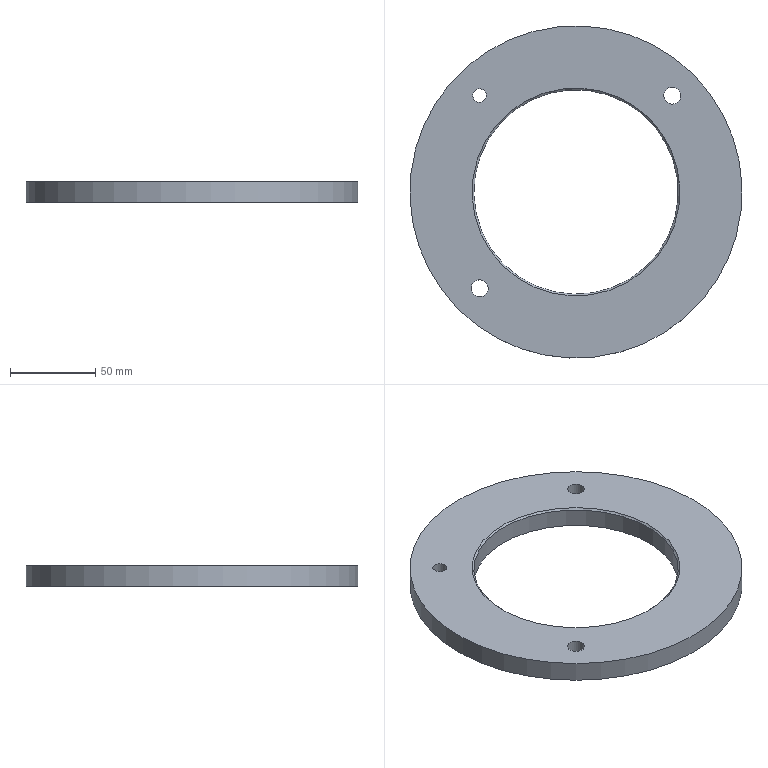Component | NX | CA6140-ZHUZHOU-YOUGAI | 1 solid | 8 faces | box 195 x 195 x 12 mm | volume 219983 mm3 | cylinder 5 | plane 2 | cone 1 | commonest cylinder face diameters 10 x2 195 x1 120 x1 8 x1
STEP:
#1=CARTESIAN_POINT('',(0.,0.,0.));
#2=DIRECTION('',(0.,0.,1.));
#3=DIRECTION('',(1.,0.,0.));
#4=AXIS2_PLACEMENT_3D('',#1,#2,#3);
#5=CARTESIAN_POINT('',(-43.134,-43.134,124.));
#6=VERTEX_POINT('',#5);
#7=CARTESIAN_POINT('',(0.,-0.,124.));
#8=DIRECTION('',(0.,0.,-1.));
#9=DIRECTION('',(-0.7071,-0.7071,0.));
#10=AXIS2_PLACEMENT_3D('',#7,#8,#9);
#11=CIRCLE('',#10,61.);
#12=CARTESIAN_POINT('',(0.,-0.,124.));
#13=DIRECTION('',(0.,0.,1.));
#14=DIRECTION('',(-0.7071,-0.7071,0.));
#15=AXIS2_PLACEMENT_3D('',#12,#13,#14);
#16=PLANE('',#15);
#17=CARTESIAN_POINT('',(61.,0.));
#18=CARTESIAN_POINT('',(61.,-105.655));
#19=CARTESIAN_POINT('',(-30.5,-52.828));
#20=CARTESIAN_POINT('',(-122.,-0.));
#21=CARTESIAN_POINT('',(-30.5,52.828));
#22=CARTESIAN_POINT('',(61.,105.655));
#23=CARTESIAN_POINT('',(61.,0.));
#24=(BOUNDED_CURVE()B_SPLINE_CURVE(2,(#17,#18,#19,#20,#21,#22,#23),.UNSPECIFIED.,.T.,.F.)B_SPLINE_CURVE_WITH_KNOTS((1,2,2,2,2,1),(-2.094,0.,2.094,4.189,6.283,8.378),.UNSPECIFIED.)CURVE()GEOMETRIC_REPRESENTATION_ITEM()RATIONAL_B_SPLINE_CURVE((1.,0.5,1.,0.5,1.,0.5,1.))REPRESENTATION_ITEM(''));
#25=(GEOMETRIC_REPRESENTATION_CONTEXT(2)PARAMETRIC_REPRESENTATION_CONTEXT()REPRESENTATION_CONTEXT('',''));
#26=DEFINITIONAL_REPRESENTATION('',(#24),#25);
#27=PCURVE('',#16,#26);
#28=CARTESIAN_POINT('',(0.,-0.,123.));
#29=DIRECTION('',(0.,0.,1.));
#30=DIRECTION('',(-0.7071,-0.7071,0.));
#31=AXIS2_PLACEMENT_3D('',#28,#29,#30);
#32=CONICAL_SURFACE('',#31,60.,0.7854);
#33=CARTESIAN_POINT('',(6.283,1.));
#34=DIRECTION('',(-1.,0.));
#35=VECTOR('',#34,1.);
#36=LINE('',#33,#35);
#37=(GEOMETRIC_REPRESENTATION_CONTEXT(2)PARAMETRIC_REPRESENTATION_CONTEXT()REPRESENTATION_CONTEXT('',''));
#38=DEFINITIONAL_REPRESENTATION('',(#36),#37);
#39=PCURVE('',#32,#38);
#40=SURFACE_CURVE('',#11,(#27,#39),.PCURVE_S1.);
#41=EDGE_CURVE('',#6,#6,#40,.T.);
#42=ORIENTED_EDGE('',*,*,#41,.T.);
#43=EDGE_LOOP('',(#42));
#44=FACE_BOUND('',#43,.T.);
#45=CARTESIAN_POINT('',(53.033,53.033,124.));
#46=VERTEX_POINT('',#45);
#47=CARTESIAN_POINT('',(56.569,56.569,124.));
#48=DIRECTION('',(0.,0.,-1.));
#49=DIRECTION('',(-0.7071,-0.7071,0.));
#50=AXIS2_PLACEMENT_3D('',#47,#48,#49);
#51=CIRCLE('',#50,5.);
#52=CARTESIAN_POINT('',(-75.,-0.));
#53=CARTESIAN_POINT('',(-75.,-8.66));
#54=CARTESIAN_POINT('',(-82.5,-4.33));
#55=CARTESIAN_POINT('',(-90.,-0.));
#56=CARTESIAN_POINT('',(-82.5,4.33));
#57=CARTESIAN_POINT('',(-75.,8.66));
#58=CARTESIAN_POINT('',(-75.,-0.));
#59=(BOUNDED_CURVE()B_SPLINE_CURVE(2,(#52,#53,#54,#55,#56,#57,#58),.UNSPECIFIED.,.T.,.F.)B_SPLINE_CURVE_WITH_KNOTS((1,2,2,2,2,1),(-2.094,0.,2.094,4.189,6.283,8.378),.UNSPECIFIED.)CURVE()GEOMETRIC_REPRESENTATION_ITEM()RATIONAL_B_SPLINE_CURVE((1.,0.5,1.,0.5,1.,0.5,1.))REPRESENTATION_ITEM(''));
#60=(GEOMETRIC_REPRESENTATION_CONTEXT(2)PARAMETRIC_REPRESENTATION_CONTEXT()REPRESENTATION_CONTEXT('',''));
#61=DEFINITIONAL_REPRESENTATION('',(#59),#60);
#62=PCURVE('',#16,#61);
#63=CARTESIAN_POINT('',(56.569,56.569,124.));
#64=DIRECTION('',(0.,0.,-1.));
#65=DIRECTION('',(0.7071,0.7071,0.));
#66=AXIS2_PLACEMENT_3D('',#63,#64,#65);
#67=CYLINDRICAL_SURFACE('',#66,5.);
#68=CARTESIAN_POINT('',(3.142,0.));
#69=DIRECTION('',(1.,0.));
#70=VECTOR('',#69,1.);
#71=LINE('',#68,#70);
#72=(GEOMETRIC_REPRESENTATION_CONTEXT(2)PARAMETRIC_REPRESENTATION_CONTEXT()REPRESENTATION_CONTEXT('',''));
#73=DEFINITIONAL_REPRESENTATION('',(#71),#72);
#74=PCURVE('',#67,#73);
#75=SURFACE_CURVE('',#51,(#62,#74),.PCURVE_S1.);
#76=EDGE_CURVE('',#46,#46,#75,.T.);
#77=ORIENTED_EDGE('',*,*,#76,.T.);
#78=EDGE_LOOP('',(#77));
#79=FACE_BOUND('',#78,.T.);
#80=CARTESIAN_POINT('',(-60.104,-60.104,124.));
#81=VERTEX_POINT('',#80);
#82=CARTESIAN_POINT('',(-56.569,-56.569,124.));
#83=DIRECTION('',(0.,0.,1.));
#84=DIRECTION('',(-0.7071,-0.7071,0.));
#85=AXIS2_PLACEMENT_3D('',#82,#83,#84);
#86=CIRCLE('',#85,5.);
#87=CARTESIAN_POINT('',(80.,-0.));
#88=DIRECTION('',(1.,0.));
#89=AXIS2_PLACEMENT_2D('',#87,#88);
#90=CIRCLE('',#89,5.);
#91=(GEOMETRIC_REPRESENTATION_CONTEXT(2)PARAMETRIC_REPRESENTATION_CONTEXT()REPRESENTATION_CONTEXT('',''));
#92=DEFINITIONAL_REPRESENTATION('',(#90),#91);
#93=PCURVE('',#16,#92);
#94=CARTESIAN_POINT('',(-56.569,-56.569,124.));
#95=DIRECTION('',(0.,0.,-1.));
#96=DIRECTION('',(0.7071,0.7071,0.));
#97=AXIS2_PLACEMENT_3D('',#94,#95,#96);
#98=CYLINDRICAL_SURFACE('',#97,5.);
#99=CARTESIAN_POINT('',(9.425,0.));
#100=DIRECTION('',(-1.,0.));
#101=VECTOR('',#100,1.);
#102=LINE('',#99,#101);
#103=(GEOMETRIC_REPRESENTATION_CONTEXT(2)PARAMETRIC_REPRESENTATION_CONTEXT()REPRESENTATION_CONTEXT('',''));
#104=DEFINITIONAL_REPRESENTATION('',(#102),#103);
#105=PCURVE('',#98,#104);
#106=SURFACE_CURVE('',#86,(#93,#105),.PCURVE_S1.);
#107=EDGE_CURVE('',#81,#81,#106,.T.);
#108=ORIENTED_EDGE('',*,*,#107,.F.);
#109=EDGE_LOOP('',(#108));
#110=FACE_BOUND('',#109,.T.);
#111=CARTESIAN_POINT('',(68.943,68.943,124.));
#112=VERTEX_POINT('',#111);
#113=CARTESIAN_POINT('',(-68.943,-68.943,124.));
#114=VERTEX_POINT('',#113);
#115=CARTESIAN_POINT('',(0.,-0.,124.));
#116=DIRECTION('',(0.,0.,-1.));
#117=DIRECTION('',(0.7071,0.7071,0.));
#118=AXIS2_PLACEMENT_3D('',#115,#116,#117);
#119=CIRCLE('',#118,97.5);
#120=CARTESIAN_POINT('',(-97.5,0.));
#121=CARTESIAN_POINT('',(-97.5,168.875));
#122=CARTESIAN_POINT('',(48.75,84.437));
#123=CARTESIAN_POINT('',(195.,0.));
#124=CARTESIAN_POINT('',(48.75,-84.437));
#125=CARTESIAN_POINT('',(-97.5,-168.875));
#126=CARTESIAN_POINT('',(-97.5,0.));
#127=(BOUNDED_CURVE()B_SPLINE_CURVE(2,(#120,#121,#122,#123,#124,#125,#126),.UNSPECIFIED.,.T.,.F.)B_SPLINE_CURVE_WITH_KNOTS((1,2,2,2,2,1),(-2.094,0.,2.094,4.189,6.283,8.378),.UNSPECIFIED.)CURVE()GEOMETRIC_REPRESENTATION_ITEM()RATIONAL_B_SPLINE_CURVE((1.,0.5,1.,0.5,1.,0.5,1.))REPRESENTATION_ITEM(''));
#128=(GEOMETRIC_REPRESENTATION_CONTEXT(2)PARAMETRIC_REPRESENTATION_CONTEXT()REPRESENTATION_CONTEXT('',''));
#129=DEFINITIONAL_REPRESENTATION('',(#127),#128);
#130=PCURVE('',#16,#129);
#131=CARTESIAN_POINT('',(0.,-0.,112.));
#132=DIRECTION('',(0.,0.,1.));
#133=DIRECTION('',(-0.7071,-0.7071,0.));
#134=AXIS2_PLACEMENT_3D('',#131,#132,#133);
#135=CYLINDRICAL_SURFACE('',#134,97.5);
#136=CARTESIAN_POINT('',(3.142,12.));
#137=DIRECTION('',(-1.,0.));
#138=VECTOR('',#137,1.);
#139=LINE('',#136,#138);
#140=(GEOMETRIC_REPRESENTATION_CONTEXT(2)PARAMETRIC_REPRESENTATION_CONTEXT()REPRESENTATION_CONTEXT('',''));
#141=DEFINITIONAL_REPRESENTATION('',(#139),#140);
#142=PCURVE('',#135,#141);
#143=SURFACE_CURVE('',#119,(#130,#142),.PCURVE_S1.);
#144=EDGE_CURVE('',#112,#114,#143,.T.);
#145=ORIENTED_EDGE('',*,*,#144,.F.);
#146=CARTESIAN_POINT('',(0.,-0.,124.));
#147=DIRECTION('',(0.,0.,-1.));
#148=DIRECTION('',(0.7071,0.7071,0.));
#149=AXIS2_PLACEMENT_3D('',#146,#147,#148);
#150=CIRCLE('',#149,97.5);
#151=CARTESIAN_POINT('',(-97.5,0.));
#152=CARTESIAN_POINT('',(-97.5,168.875));
#153=CARTESIAN_POINT('',(48.75,84.437));
#154=CARTESIAN_POINT('',(195.,0.));
#155=CARTESIAN_POINT('',(48.75,-84.437));
#156=CARTESIAN_POINT('',(-97.5,-168.875));
#157=CARTESIAN_POINT('',(-97.5,0.));
#158=(BOUNDED_CURVE()B_SPLINE_CURVE(2,(#151,#152,#153,#154,#155,#156,#157),.UNSPECIFIED.,.T.,.F.)B_SPLINE_CURVE_WITH_KNOTS((1,2,2,2,2,1),(-2.094,0.,2.094,4.189,6.283,8.378),.UNSPECIFIED.)CURVE()GEOMETRIC_REPRESENTATION_ITEM()RATIONAL_B_SPLINE_CURVE((1.,0.5,1.,0.5,1.,0.5,1.))REPRESENTATION_ITEM(''));
#159=(GEOMETRIC_REPRESENTATION_CONTEXT(2)PARAMETRIC_REPRESENTATION_CONTEXT()REPRESENTATION_CONTEXT('',''));
#160=DEFINITIONAL_REPRESENTATION('',(#158),#159);
#161=PCURVE('',#16,#160);
#162=CARTESIAN_POINT('',(9.425,12.));
#163=DIRECTION('',(-1.,0.));
#164=VECTOR('',#163,1.);
#165=LINE('',#162,#164);
#166=(GEOMETRIC_REPRESENTATION_CONTEXT(2)PARAMETRIC_REPRESENTATION_CONTEXT()REPRESENTATION_CONTEXT('',''));
#167=DEFINITIONAL_REPRESENTATION('',(#165),#166);
#168=PCURVE('',#135,#167);
#169=SURFACE_CURVE('',#150,(#161,#168),.PCURVE_S1.);
#170=EDGE_CURVE('',#114,#112,#169,.T.);
#171=ORIENTED_EDGE('',*,*,#170,.F.);
#172=EDGE_LOOP('',(#145,#171));
#173=FACE_BOUND('',#172,.T.);
#174=CARTESIAN_POINT('',(-59.397,53.74,124.));
#175=VERTEX_POINT('',#174);
#176=CARTESIAN_POINT('',(-56.569,56.569,124.));
#177=DIRECTION('',(0.,0.,-1.));
#178=DIRECTION('',(-0.7071,-0.7071,0.));
#179=AXIS2_PLACEMENT_3D('',#176,#177,#178);
#180=CIRCLE('',#179,4.);
#181=CARTESIAN_POINT('',(4.,-80.));
#182=CARTESIAN_POINT('',(4.,-86.928));
#183=CARTESIAN_POINT('',(-2.,-83.464));
#184=CARTESIAN_POINT('',(-8.,-80.));
#185=CARTESIAN_POINT('',(-2.,-76.536));
#186=CARTESIAN_POINT('',(4.,-73.072));
#187=CARTESIAN_POINT('',(4.,-80.));
#188=(BOUNDED_CURVE()B_SPLINE_CURVE(2,(#181,#182,#183,#184,#185,#186,#187),.UNSPECIFIED.,.T.,.F.)B_SPLINE_CURVE_WITH_KNOTS((1,2,2,2,2,1),(-2.094,0.,2.094,4.189,6.283,8.378),.UNSPECIFIED.)CURVE()GEOMETRIC_REPRESENTATION_ITEM()RATIONAL_B_SPLINE_CURVE((1.,0.5,1.,0.5,1.,0.5,1.))REPRESENTATION_ITEM(''));
#189=(GEOMETRIC_REPRESENTATION_CONTEXT(2)PARAMETRIC_REPRESENTATION_CONTEXT()REPRESENTATION_CONTEXT('',''));
#190=DEFINITIONAL_REPRESENTATION('',(#188),#189);
#191=PCURVE('',#16,#190);
#192=CARTESIAN_POINT('',(-56.569,56.569,124.));
#193=DIRECTION('',(0.,0.,-1.));
#194=DIRECTION('',(0.7071,0.7071,0.));
#195=AXIS2_PLACEMENT_3D('',#192,#193,#194);
#196=CYLINDRICAL_SURFACE('',#195,4.);
#197=CARTESIAN_POINT('',(3.142,0.));
#198=DIRECTION('',(1.,0.));
#199=VECTOR('',#198,1.);
#200=LINE('',#197,#199);
#201=(GEOMETRIC_REPRESENTATION_CONTEXT(2)PARAMETRIC_REPRESENTATION_CONTEXT()REPRESENTATION_CONTEXT('',''));
#202=DEFINITIONAL_REPRESENTATION('',(#200),#201);
#203=PCURVE('',#196,#202);
#204=SURFACE_CURVE('',#180,(#191,#203),.PCURVE_S1.);
#205=EDGE_CURVE('',#175,#175,#204,.T.);
#206=ORIENTED_EDGE('',*,*,#205,.T.);
#207=EDGE_LOOP('',(#206));
#208=FACE_BOUND('',#207,.T.);
#209=ADVANCED_FACE('',(#44,#79,#110,#173,#208),#16,.T.);
#210=CARTESIAN_POINT('',(-59.397,53.74,112.));
#211=VERTEX_POINT('',#210);
#212=CARTESIAN_POINT('',(-56.569,56.569,112.));
#213=DIRECTION('',(0.,0.,-1.));
#214=DIRECTION('',(-0.7071,-0.7071,0.));
#215=AXIS2_PLACEMENT_3D('',#212,#213,#214);
#216=CIRCLE('',#215,4.);
#217=CARTESIAN_POINT('',(0.,-0.,112.));
#218=DIRECTION('',(0.,0.,-1.));
#219=DIRECTION('',(0.7071,0.7071,0.));
#220=AXIS2_PLACEMENT_3D('',#217,#218,#219);
#221=PLANE('',#220);
#222=CARTESIAN_POINT('',(0.,-80.));
#223=DIRECTION('',(-1.,0.));
#224=AXIS2_PLACEMENT_2D('',#222,#223);
#225=CIRCLE('',#224,4.);
#226=(GEOMETRIC_REPRESENTATION_CONTEXT(2)PARAMETRIC_REPRESENTATION_CONTEXT()REPRESENTATION_CONTEXT('',''));
#227=DEFINITIONAL_REPRESENTATION('',(#225),#226);
#228=PCURVE('',#221,#227);
#229=CARTESIAN_POINT('',(3.142,12.));
#230=DIRECTION('',(1.,0.));
#231=VECTOR('',#230,1.);
#232=LINE('',#229,#231);
#233=(GEOMETRIC_REPRESENTATION_CONTEXT(2)PARAMETRIC_REPRESENTATION_CONTEXT()REPRESENTATION_CONTEXT('',''));
#234=DEFINITIONAL_REPRESENTATION('',(#232),#233);
#235=PCURVE('',#196,#234);
#236=SURFACE_CURVE('',#216,(#228,#235),.PCURVE_S1.);
#237=EDGE_CURVE('',#211,#211,#236,.T.);
#238=ORIENTED_EDGE('',*,*,#237,.F.);
#239=EDGE_LOOP('',(#238));
#240=FACE_BOUND('',#239,.T.);
#241=CARTESIAN_POINT('',(53.033,53.033,112.));
#242=VERTEX_POINT('',#241);
#243=CARTESIAN_POINT('',(56.569,56.569,112.));
#244=DIRECTION('',(0.,0.,-1.));
#245=DIRECTION('',(-0.7071,-0.7071,0.));
#246=AXIS2_PLACEMENT_3D('',#243,#244,#245);
#247=CIRCLE('',#246,5.);
#248=CARTESIAN_POINT('',(80.,-0.));
#249=DIRECTION('',(-1.,0.));
#250=AXIS2_PLACEMENT_2D('',#248,#249);
#251=CIRCLE('',#250,5.);
#252=(GEOMETRIC_REPRESENTATION_CONTEXT(2)PARAMETRIC_REPRESENTATION_CONTEXT()REPRESENTATION_CONTEXT('',''));
#253=DEFINITIONAL_REPRESENTATION('',(#251),#252);
#254=PCURVE('',#221,#253);
#255=CARTESIAN_POINT('',(3.142,12.));
#256=DIRECTION('',(1.,0.));
#257=VECTOR('',#256,1.);
#258=LINE('',#255,#257);
#259=(GEOMETRIC_REPRESENTATION_CONTEXT(2)PARAMETRIC_REPRESENTATION_CONTEXT()REPRESENTATION_CONTEXT('',''));
#260=DEFINITIONAL_REPRESENTATION('',(#258),#259);
#261=PCURVE('',#67,#260);
#262=SURFACE_CURVE('',#247,(#254,#261),.PCURVE_S1.);
#263=EDGE_CURVE('',#242,#242,#262,.T.);
#264=ORIENTED_EDGE('',*,*,#263,.F.);
#265=EDGE_LOOP('',(#264));
#266=FACE_BOUND('',#265,.T.);
#267=CARTESIAN_POINT('',(-68.943,-68.943,112.));
#268=VERTEX_POINT('',#267);
#269=CARTESIAN_POINT('',(0.,-0.,112.));
#270=DIRECTION('',(0.,0.,1.));
#271=DIRECTION('',(-0.7071,-0.7071,0.));
#272=AXIS2_PLACEMENT_3D('',#269,#270,#271);
#273=CIRCLE('',#272,97.5);
#274=CARTESIAN_POINT('',(-97.5,0.));
#275=CARTESIAN_POINT('',(-97.5,168.875));
#276=CARTESIAN_POINT('',(48.75,84.437));
#277=CARTESIAN_POINT('',(195.,0.));
#278=CARTESIAN_POINT('',(48.75,-84.437));
#279=CARTESIAN_POINT('',(-97.5,-168.875));
#280=CARTESIAN_POINT('',(-97.5,0.));
#281=(BOUNDED_CURVE()B_SPLINE_CURVE(2,(#274,#275,#276,#277,#278,#279,#280),.UNSPECIFIED.,.T.,.F.)B_SPLINE_CURVE_WITH_KNOTS((1,2,2,2,2,1),(-2.094,0.,2.094,4.189,6.283,8.378),.UNSPECIFIED.)CURVE()GEOMETRIC_REPRESENTATION_ITEM()RATIONAL_B_SPLINE_CURVE((1.,0.5,1.,0.5,1.,0.5,1.))REPRESENTATION_ITEM(''));
#282=(GEOMETRIC_REPRESENTATION_CONTEXT(2)PARAMETRIC_REPRESENTATION_CONTEXT()REPRESENTATION_CONTEXT('',''));
#283=DEFINITIONAL_REPRESENTATION('',(#281),#282);
#284=PCURVE('',#221,#283);
#285=CARTESIAN_POINT('',(0.,0.));
#286=DIRECTION('',(1.,0.));
#287=VECTOR('',#286,1.);
#288=LINE('',#285,#287);
#289=(GEOMETRIC_REPRESENTATION_CONTEXT(2)PARAMETRIC_REPRESENTATION_CONTEXT()REPRESENTATION_CONTEXT('',''));
#290=DEFINITIONAL_REPRESENTATION('',(#288),#289);
#291=PCURVE('',#135,#290);
#292=SURFACE_CURVE('',#273,(#284,#291),.PCURVE_S1.);
#293=EDGE_CURVE('',#268,#268,#292,.T.);
#294=ORIENTED_EDGE('',*,*,#293,.F.);
#295=EDGE_LOOP('',(#294));
#296=FACE_BOUND('',#295,.T.);
#297=CARTESIAN_POINT('',(-42.426,-42.426,112.));
#298=VERTEX_POINT('',#297);
#299=CARTESIAN_POINT('',(0.,-0.,112.));
#300=DIRECTION('',(0.,0.,1.));
#301=DIRECTION('',(-0.7071,-0.7071,0.));
#302=AXIS2_PLACEMENT_3D('',#299,#300,#301);
#303=CIRCLE('',#302,60.);
#304=CARTESIAN_POINT('',(-60.,0.));
#305=CARTESIAN_POINT('',(-60.,103.923));
#306=CARTESIAN_POINT('',(30.,51.962));
#307=CARTESIAN_POINT('',(120.,0.));
#308=CARTESIAN_POINT('',(30.,-51.962));
#309=CARTESIAN_POINT('',(-60.,-103.923));
#310=CARTESIAN_POINT('',(-60.,0.));
#311=(BOUNDED_CURVE()B_SPLINE_CURVE(2,(#304,#305,#306,#307,#308,#309,#310),.UNSPECIFIED.,.T.,.F.)B_SPLINE_CURVE_WITH_KNOTS((1,2,2,2,2,1),(-2.094,0.,2.094,4.189,6.283,8.378),.UNSPECIFIED.)CURVE()GEOMETRIC_REPRESENTATION_ITEM()RATIONAL_B_SPLINE_CURVE((1.,0.5,1.,0.5,1.,0.5,1.))REPRESENTATION_ITEM(''));
#312=(GEOMETRIC_REPRESENTATION_CONTEXT(2)PARAMETRIC_REPRESENTATION_CONTEXT()REPRESENTATION_CONTEXT('',''));
#313=DEFINITIONAL_REPRESENTATION('',(#311),#312);
#314=PCURVE('',#221,#313);
#315=CARTESIAN_POINT('',(0.,-0.,112.));
#316=DIRECTION('',(0.,0.,1.));
#317=DIRECTION('',(-0.7071,-0.7071,0.));
#318=AXIS2_PLACEMENT_3D('',#315,#316,#317);
#319=CYLINDRICAL_SURFACE('',#318,60.);
#320=CARTESIAN_POINT('',(0.,0.));
#321=DIRECTION('',(1.,0.));
#322=VECTOR('',#321,1.);
#323=LINE('',#320,#322);
#324=(GEOMETRIC_REPRESENTATION_CONTEXT(2)PARAMETRIC_REPRESENTATION_CONTEXT()REPRESENTATION_CONTEXT('',''));
#325=DEFINITIONAL_REPRESENTATION('',(#323),#324);
#326=PCURVE('',#319,#325);
#327=SURFACE_CURVE('',#303,(#314,#326),.PCURVE_S1.);
#328=EDGE_CURVE('',#298,#298,#327,.T.);
#329=ORIENTED_EDGE('',*,*,#328,.T.);
#330=EDGE_LOOP('',(#329));
#331=FACE_BOUND('',#330,.T.);
#332=CARTESIAN_POINT('',(-60.104,-60.104,112.));
#333=VERTEX_POINT('',#332);
#334=CARTESIAN_POINT('',(-56.569,-56.569,112.));
#335=DIRECTION('',(0.,0.,1.));
#336=DIRECTION('',(-0.7071,-0.7071,0.));
#337=AXIS2_PLACEMENT_3D('',#334,#335,#336);
#338=CIRCLE('',#337,5.);
#339=CARTESIAN_POINT('',(-85.,-0.));
#340=CARTESIAN_POINT('',(-85.,8.66));
#341=CARTESIAN_POINT('',(-77.5,4.33));
#342=CARTESIAN_POINT('',(-70.,-0.));
#343=CARTESIAN_POINT('',(-77.5,-4.33));
#344=CARTESIAN_POINT('',(-85.,-8.66));
#345=CARTESIAN_POINT('',(-85.,-0.));
#346=(BOUNDED_CURVE()B_SPLINE_CURVE(2,(#339,#340,#341,#342,#343,#344,#345),.UNSPECIFIED.,.T.,.F.)B_SPLINE_CURVE_WITH_KNOTS((1,2,2,2,2,1),(-2.094,0.,2.094,4.189,6.283,8.378),.UNSPECIFIED.)CURVE()GEOMETRIC_REPRESENTATION_ITEM()RATIONAL_B_SPLINE_CURVE((1.,0.5,1.,0.5,1.,0.5,1.))REPRESENTATION_ITEM(''));
#347=(GEOMETRIC_REPRESENTATION_CONTEXT(2)PARAMETRIC_REPRESENTATION_CONTEXT()REPRESENTATION_CONTEXT('',''));
#348=DEFINITIONAL_REPRESENTATION('',(#346),#347);
#349=PCURVE('',#221,#348);
#350=CARTESIAN_POINT('',(9.425,12.));
#351=DIRECTION('',(-1.,0.));
#352=VECTOR('',#351,1.);
#353=LINE('',#350,#352);
#354=(GEOMETRIC_REPRESENTATION_CONTEXT(2)PARAMETRIC_REPRESENTATION_CONTEXT()REPRESENTATION_CONTEXT('',''));
#355=DEFINITIONAL_REPRESENTATION('',(#353),#354);
#356=PCURVE('',#98,#355);
#357=SURFACE_CURVE('',#338,(#349,#356),.PCURVE_S1.);
#358=EDGE_CURVE('',#333,#333,#357,.T.);
#359=ORIENTED_EDGE('',*,*,#358,.T.);
#360=EDGE_LOOP('',(#359));
#361=FACE_BOUND('',#360,.T.);
#362=ADVANCED_FACE('',(#240,#266,#296,#331,#361),#221,.T.);
#363=ORIENTED_EDGE('',*,*,#144,.T.);
#364=CARTESIAN_POINT('',(-68.943,-68.943,112.));
#365=CARTESIAN_POINT('',(-68.943,-68.943,124.));
#366=B_SPLINE_CURVE_WITH_KNOTS('',1,(#364,#365),.UNSPECIFIED.,.F.,.F.,(2,2),(0.,12.),.PIECEWISE_BEZIER_KNOTS.);
#367=CARTESIAN_POINT('',(0.,0.));
#368=DIRECTION('',(0.,1.));
#369=VECTOR('',#368,1.);
#370=LINE('',#367,#369);
#371=(GEOMETRIC_REPRESENTATION_CONTEXT(2)PARAMETRIC_REPRESENTATION_CONTEXT()REPRESENTATION_CONTEXT('',''));
#372=DEFINITIONAL_REPRESENTATION('',(#370),#371);
#373=PCURVE('',#135,#372);
#374=CARTESIAN_POINT('',(6.283,0.));
#375=DIRECTION('',(0.,1.));
#376=VECTOR('',#375,1.);
#377=LINE('',#374,#376);
#378=(GEOMETRIC_REPRESENTATION_CONTEXT(2)PARAMETRIC_REPRESENTATION_CONTEXT()REPRESENTATION_CONTEXT('',''));
#379=DEFINITIONAL_REPRESENTATION('',(#377),#378);
#380=PCURVE('',#135,#379);
#381=SEAM_CURVE('',#366,(#373,#380),.PCURVE_S1.);
#382=EDGE_CURVE('',#268,#114,#381,.T.);
#383=ORIENTED_EDGE('',*,*,#382,.F.);
#384=ORIENTED_EDGE('',*,*,#293,.T.);
#385=ORIENTED_EDGE('',*,*,#382,.T.);
#386=ORIENTED_EDGE('',*,*,#170,.T.);
#387=EDGE_LOOP('',(#363,#383,#384,#385,#386));
#388=FACE_BOUND('',#387,.T.);
#389=ADVANCED_FACE('',(#388),#135,.T.);
#390=CARTESIAN_POINT('',(-42.426,-42.426,123.));
#391=VERTEX_POINT('',#390);
#392=CARTESIAN_POINT('',(0.,-0.,123.));
#393=DIRECTION('',(0.,0.,1.));
#394=DIRECTION('',(-0.7071,-0.7071,0.));
#395=AXIS2_PLACEMENT_3D('',#392,#393,#394);
#396=CIRCLE('',#395,60.);
#397=CARTESIAN_POINT('',(0.,11.));
#398=DIRECTION('',(1.,0.));
#399=VECTOR('',#398,1.);
#400=LINE('',#397,#399);
#401=(GEOMETRIC_REPRESENTATION_CONTEXT(2)PARAMETRIC_REPRESENTATION_CONTEXT()REPRESENTATION_CONTEXT('',''));
#402=DEFINITIONAL_REPRESENTATION('',(#400),#401);
#403=PCURVE('',#319,#402);
#404=CARTESIAN_POINT('',(0.,0.));
#405=DIRECTION('',(1.,0.));
#406=VECTOR('',#405,1.);
#407=LINE('',#404,#406);
#408=(GEOMETRIC_REPRESENTATION_CONTEXT(2)PARAMETRIC_REPRESENTATION_CONTEXT()REPRESENTATION_CONTEXT('',''));
#409=DEFINITIONAL_REPRESENTATION('',(#407),#408);
#410=PCURVE('',#32,#409);
#411=SURFACE_CURVE('',#396,(#403,#410),.PCURVE_S1.);
#412=EDGE_CURVE('',#391,#391,#411,.T.);
#413=ORIENTED_EDGE('',*,*,#412,.F.);
#414=CARTESIAN_POINT('',(-42.426,-42.426,112.));
#415=CARTESIAN_POINT('',(-42.426,-42.426,123.));
#416=B_SPLINE_CURVE_WITH_KNOTS('',1,(#414,#415),.UNSPECIFIED.,.F.,.F.,(2,2),(0.,11.),.PIECEWISE_BEZIER_KNOTS.);
#417=CARTESIAN_POINT('',(0.,0.));
#418=DIRECTION('',(0.,1.));
#419=VECTOR('',#418,1.);
#420=LINE('',#417,#419);
#421=(GEOMETRIC_REPRESENTATION_CONTEXT(2)PARAMETRIC_REPRESENTATION_CONTEXT()REPRESENTATION_CONTEXT('',''));
#422=DEFINITIONAL_REPRESENTATION('',(#420),#421);
#423=PCURVE('',#319,#422);
#424=CARTESIAN_POINT('',(6.283,0.));
#425=DIRECTION('',(0.,1.));
#426=VECTOR('',#425,1.);
#427=LINE('',#424,#426);
#428=(GEOMETRIC_REPRESENTATION_CONTEXT(2)PARAMETRIC_REPRESENTATION_CONTEXT()REPRESENTATION_CONTEXT('',''));
#429=DEFINITIONAL_REPRESENTATION('',(#427),#428);
#430=PCURVE('',#319,#429);
#431=SEAM_CURVE('',#416,(#423,#430),.PCURVE_S1.);
#432=EDGE_CURVE('',#298,#391,#431,.T.);
#433=ORIENTED_EDGE('',*,*,#432,.F.);
#434=ORIENTED_EDGE('',*,*,#328,.T.);
#435=ORIENTED_EDGE('',*,*,#432,.T.);
#436=EDGE_LOOP('',(#413,#433,#434,#435));
#437=FACE_BOUND('',#436,.F.);
#438=ADVANCED_FACE('',(#437),#319,.F.);
#439=ORIENTED_EDGE('',*,*,#107,.F.);
#440=CARTESIAN_POINT('',(-60.104,-60.104,124.));
#441=CARTESIAN_POINT('',(-60.104,-60.104,112.));
#442=B_SPLINE_CURVE_WITH_KNOTS('',1,(#440,#441),.UNSPECIFIED.,.F.,.F.,(2,2),(0.,12.),.PIECEWISE_BEZIER_KNOTS.);
#443=CARTESIAN_POINT('',(9.425,0.));
#444=DIRECTION('',(0.,1.));
#445=VECTOR('',#444,1.);
#446=LINE('',#443,#445);
#447=(GEOMETRIC_REPRESENTATION_CONTEXT(2)PARAMETRIC_REPRESENTATION_CONTEXT()REPRESENTATION_CONTEXT('',''));
#448=DEFINITIONAL_REPRESENTATION('',(#446),#447);
#449=PCURVE('',#98,#448);
#450=CARTESIAN_POINT('',(3.142,0.));
#451=DIRECTION('',(0.,1.));
#452=VECTOR('',#451,1.);
#453=LINE('',#450,#452);
#454=(GEOMETRIC_REPRESENTATION_CONTEXT(2)PARAMETRIC_REPRESENTATION_CONTEXT()REPRESENTATION_CONTEXT('',''));
#455=DEFINITIONAL_REPRESENTATION('',(#453),#454);
#456=PCURVE('',#98,#455);
#457=SEAM_CURVE('',#442,(#449,#456),.PCURVE_S1.);
#458=EDGE_CURVE('',#81,#333,#457,.T.);
#459=ORIENTED_EDGE('',*,*,#458,.T.);
#460=ORIENTED_EDGE('',*,*,#358,.T.);
#461=ORIENTED_EDGE('',*,*,#458,.F.);
#462=EDGE_LOOP('',(#439,#459,#460,#461));
#463=FACE_BOUND('',#462,.F.);
#464=ADVANCED_FACE('',(#463),#98,.F.);
#465=ORIENTED_EDGE('',*,*,#76,.T.);
#466=CARTESIAN_POINT('',(53.033,53.033,124.));
#467=CARTESIAN_POINT('',(53.033,53.033,112.));
#468=B_SPLINE_CURVE_WITH_KNOTS('',1,(#466,#467),.UNSPECIFIED.,.F.,.F.,(2,2),(0.,12.),.PIECEWISE_BEZIER_KNOTS.);
#469=CARTESIAN_POINT('',(9.425,0.));
#470=DIRECTION('',(0.,1.));
#471=VECTOR('',#470,1.);
#472=LINE('',#469,#471);
#473=(GEOMETRIC_REPRESENTATION_CONTEXT(2)PARAMETRIC_REPRESENTATION_CONTEXT()REPRESENTATION_CONTEXT('',''));
#474=DEFINITIONAL_REPRESENTATION('',(#472),#473);
#475=PCURVE('',#67,#474);
#476=CARTESIAN_POINT('',(3.142,0.));
#477=DIRECTION('',(0.,1.));
#478=VECTOR('',#477,1.);
#479=LINE('',#476,#478);
#480=(GEOMETRIC_REPRESENTATION_CONTEXT(2)PARAMETRIC_REPRESENTATION_CONTEXT()REPRESENTATION_CONTEXT('',''));
#481=DEFINITIONAL_REPRESENTATION('',(#479),#480);
#482=PCURVE('',#67,#481);
#483=SEAM_CURVE('',#468,(#475,#482),.PCURVE_S1.);
#484=EDGE_CURVE('',#46,#242,#483,.T.);
#485=ORIENTED_EDGE('',*,*,#484,.T.);
#486=ORIENTED_EDGE('',*,*,#263,.F.);
#487=ORIENTED_EDGE('',*,*,#484,.F.);
#488=EDGE_LOOP('',(#465,#485,#486,#487));
#489=FACE_BOUND('',#488,.F.);
#490=ADVANCED_FACE('',(#489),#67,.F.);
#491=ORIENTED_EDGE('',*,*,#205,.T.);
#492=CARTESIAN_POINT('',(-59.397,53.74,124.));
#493=CARTESIAN_POINT('',(-59.397,53.74,112.));
#494=B_SPLINE_CURVE_WITH_KNOTS('',1,(#492,#493),.UNSPECIFIED.,.F.,.F.,(2,2),(0.,12.),.PIECEWISE_BEZIER_KNOTS.);
#495=CARTESIAN_POINT('',(9.425,0.));
#496=DIRECTION('',(0.,1.));
#497=VECTOR('',#496,1.);
#498=LINE('',#495,#497);
#499=(GEOMETRIC_REPRESENTATION_CONTEXT(2)PARAMETRIC_REPRESENTATION_CONTEXT()REPRESENTATION_CONTEXT('',''));
#500=DEFINITIONAL_REPRESENTATION('',(#498),#499);
#501=PCURVE('',#196,#500);
#502=CARTESIAN_POINT('',(3.142,0.));
#503=DIRECTION('',(0.,1.));
#504=VECTOR('',#503,1.);
#505=LINE('',#502,#504);
#506=(GEOMETRIC_REPRESENTATION_CONTEXT(2)PARAMETRIC_REPRESENTATION_CONTEXT()REPRESENTATION_CONTEXT('',''));
#507=DEFINITIONAL_REPRESENTATION('',(#505),#506);
#508=PCURVE('',#196,#507);
#509=SEAM_CURVE('',#494,(#501,#508),.PCURVE_S1.);
#510=EDGE_CURVE('',#175,#211,#509,.T.);
#511=ORIENTED_EDGE('',*,*,#510,.T.);
#512=ORIENTED_EDGE('',*,*,#237,.F.);
#513=ORIENTED_EDGE('',*,*,#510,.F.);
#514=EDGE_LOOP('',(#491,#511,#512,#513));
#515=FACE_BOUND('',#514,.F.);
#516=ADVANCED_FACE('',(#515),#196,.F.);
#517=ORIENTED_EDGE('',*,*,#41,.T.);
#518=CARTESIAN_POINT('',(-42.426,-42.426,123.));
#519=CARTESIAN_POINT('',(-43.134,-43.134,124.));
#520=B_SPLINE_CURVE_WITH_KNOTS('',1,(#518,#519),.UNSPECIFIED.,.F.,.F.,(2,2),(0.,1.414),.PIECEWISE_BEZIER_KNOTS.);
#521=CARTESIAN_POINT('',(0.,0.));
#522=DIRECTION('',(0.,1.));
#523=VECTOR('',#522,1.);
#524=LINE('',#521,#523);
#525=(GEOMETRIC_REPRESENTATION_CONTEXT(2)PARAMETRIC_REPRESENTATION_CONTEXT()REPRESENTATION_CONTEXT('',''));
#526=DEFINITIONAL_REPRESENTATION('',(#524),#525);
#527=PCURVE('',#32,#526);
#528=CARTESIAN_POINT('',(6.283,0.));
#529=DIRECTION('',(0.,1.));
#530=VECTOR('',#529,1.);
#531=LINE('',#528,#530);
#532=(GEOMETRIC_REPRESENTATION_CONTEXT(2)PARAMETRIC_REPRESENTATION_CONTEXT()REPRESENTATION_CONTEXT('',''));
#533=DEFINITIONAL_REPRESENTATION('',(#531),#532);
#534=PCURVE('',#32,#533);
#535=SEAM_CURVE('',#520,(#527,#534),.PCURVE_S1.);
#536=EDGE_CURVE('',#391,#6,#535,.T.);
#537=ORIENTED_EDGE('',*,*,#536,.F.);
#538=ORIENTED_EDGE('',*,*,#412,.T.);
#539=ORIENTED_EDGE('',*,*,#536,.T.);
#540=EDGE_LOOP('',(#517,#537,#538,#539));
#541=FACE_BOUND('',#540,.F.);
#542=ADVANCED_FACE('',(#541),#32,.F.);
#543=CLOSED_SHELL('',(#209,#362,#389,#438,#464,#490,#516,#542));
#544=MANIFOLD_SOLID_BREP('',#543);
#545=(LENGTH_UNIT()NAMED_UNIT(*)SI_UNIT(.MILLI.,.METRE.));
#546=UNCERTAINTY_MEASURE_WITH_UNIT(LENGTH_MEASURE(0.00001),#545,'','');
#547=(NAMED_UNIT(*)PLANE_ANGLE_UNIT()SI_UNIT($,.RADIAN.));
#548=(NAMED_UNIT(*)SI_UNIT($,.STERADIAN.)SOLID_ANGLE_UNIT());
#549=(GEOMETRIC_REPRESENTATION_CONTEXT(3)GLOBAL_UNCERTAINTY_ASSIGNED_CONTEXT((#546))GLOBAL_UNIT_ASSIGNED_CONTEXT((#545,#547,#548))REPRESENTATION_CONTEXT('',''));
#550=ADVANCED_BREP_SHAPE_REPRESENTATION('',(#4,#544),#549);